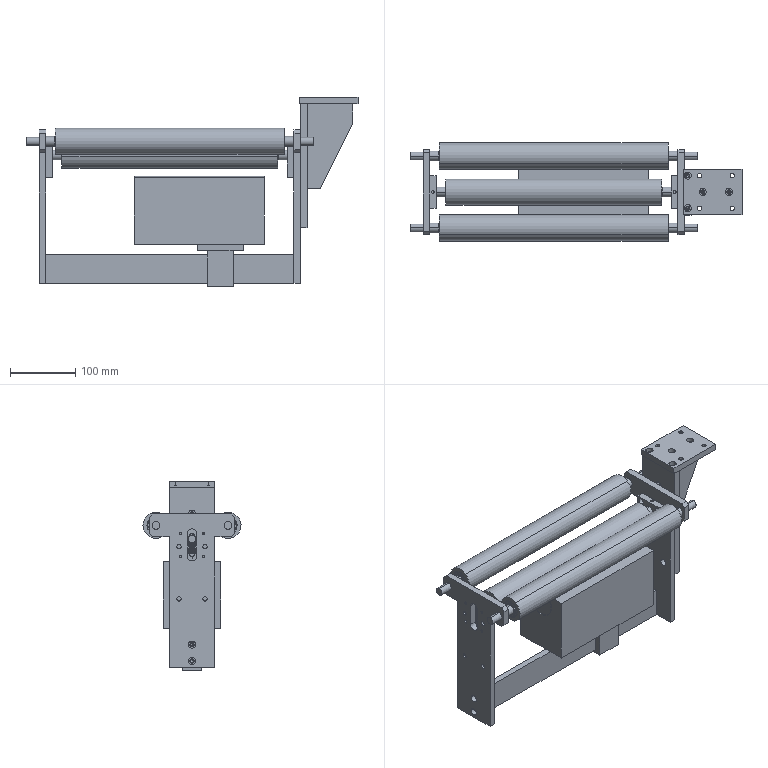Assembly | SolidWorks | mm | 25 component files | 26 solids | 1591 faces | box 508 x 150 x 290 mm | volume 3253189 mm3 | sphere 480 | cylinder 471 | plane 354 | torus 246 | cone 36 | spline 4 | commonest cylinder face diameters 25.2 x48 11 x44 6.6 x44 5 x36 4.2 x32 5.5 x32 15 x30 10 x30
Bill of materials:
01-04MarkingMachineMountingBasePlate | 1 | A3 Steel | Flat rectangular plate with eight round holes through its thickness, in three rows (3-2-3).
01-05MarkingMachineMountingVerticalPlate | 1 | A3 Steel | Thin rectangular bar or plate with six holes through its face and two blind holes drilled into one narrow end face.
01-06MarkingMachineMountingReinforcementPlate | 1 | A3 Steel | Tapered plate: one straight vertical edge, a short parallel section at the top, then an angled edge narrowing toward the bottom. Two blind holes are drilled into the top edge face.
01-07MarkingMachineDrumConnectingPlate1 | 2 | A3 Steel | T-shaped flat plate. The top crossbar has chamfered corners and a large hole at each end. The stem has a central slot with rounded ends near the top, surrounded by small holes, plus further holes lower down.
01-08MarkingMachineDrumConnectingPlate2 | 1 | A3 Steel | Long, solid rectangular bar with two blind holes drilled into one end face.
01-09MarkingMachineIdlerRollerAxis | 2 | A3 Steel | Solid round shaft with stepped ends: a long main section, a short intermediate step, and a smaller-diameter end section at each end.
01-10MarkingMachineIdlerRoller | 2 | A3 Steel | Plain, straight round tube (hollow cylinder) with uniform outside diameter.
01-11CodingRubberRollerMountingPlate | 2 | A3 Steel | Thick, nearly square block with four corner through holes, a central slot with rounded ends, and a cross hole drilled from the top edge face that meets the slot.
01-12MarkingMachinePrintingRollerAxis | 1 | A3 Steel | Long, slender round shaft with reduced-diameter ends. Each end has flat faces and a small hole drilled across it.
01-13MarkingMachinePrintingRoller | 1 | A3 Steel | Plain, straight round tube (hollow cylinder) with uniform outside diameter.
01-14MarkingMachineMountingSeatPlate | 1 | A3 Steel | Rectangular block with a long rectangular opening running through it, and four blind holes near the corners of one face.
01-15MarkingMachineMountingSeatPlate2 | 1 | A3 Steel | Flat rectangular plate with eight round holes through it: four near the corners and four further in, forming a smaller rectangle.
DK1300AInkRollerCoder | 1 | A3 Steel | Rectangular prismatic block with a full-length cylindrical feature running along its long axis just under the top face. The cylinder breaks through the top face and sticks up slightly above it. A thin gap around the cylinder suggests it is a separate rod sitting in a matching through-bore or slot.
GB_T276-94DeepGrooveBallBearing61902-2Z | 6 |  | Annular part shaped like a rolling-element bearing: a concentric outer ring and inner ring with a ring of roughly spherical elements in the annular gap between them, and a plain cylindrical bore.
OuterDiameter10WireDiameter1Height20CompressionSpring | 2 | A3 Steel | Helical coil of round-section wire, shaped like a compression spring, with a flat annular end face and evenly spaced open coils.
Mates:
1. coincident | 01-04MarkingMachineMountingBasePlate-1 face at (-13.91, 2.41, 85) dir (0, 0, -1) | 01-05MarkingMachineMountingVerticalPlate-1 face at (-56.91, -32.59, 85) dir (0, 0, 1)
2. concentric | 01-04MarkingMachineMountingBasePlate-1 face at (-51.91, -22.59, 95) dir (0, 0, 1) r 3.3 | 01-05MarkingMachineMountingVerticalPlate-1 face at (-51.91, -22.59, 85) dir (0, 0, 1) r 2.5
3. concentric | 01-04MarkingMachineMountingBasePlate-1 face at (-51.91, 27.41, 95) dir (0, 0, 1) r 3.3 | 01-05MarkingMachineMountingVerticalPlate-1 face at (-51.91, 27.41, 85) dir (0, 0, 1) r 2.5
4. coincident | 01-04MarkingMachineMountingBasePlate-1 face at (-13.91, 2.41, 85) dir (0, 0, -1) | 01-06MarkingMachineMountingReinforcementPlate-1 face at (-46.91, -2.59, 85) dir (0, 0, 1)
5. coincident | 01-05MarkingMachineMountingVerticalPlate-1 face at (-46.91, 2.41, -10) dir (1, 0, 0) | 01-06MarkingMachineMountingReinforcementPlate-1 face at (-46.91, -2.59, -45) dir (-1, 0, 0)
6. concentric | 01-05MarkingMachineMountingVerticalPlate-1 face at (-56.91, 2.41, -25) dir (-1, 0, 0) r 3.3 | 01-06MarkingMachineMountingReinforcementPlate-1 face at (-46.91, 2.41, -25) dir (-1, 0, 0) r 2.5
7. coincident | 01-05MarkingMachineMountingVerticalPlate-1 face at (-56.91, 2.41, -10) dir (-1, 0, 0) | 01-07MarkingMachineDrumConnectingPlate1-1 face at (-56.91, 2.41, 45) dir (1, 0, 0)
8. concentric | 01-07MarkingMachineDrumConnectingPlate1-1 face at (-66.91, -17.59, -5) dir (-1, 0, 0) r 5.5 | 01-05MarkingMachineMountingVerticalPlate-1 face at (-56.91, -17.59, -5) dir (-1, 0, 0) r 2.5
9. concentric | 01-05MarkingMachineMountingVerticalPlate-1 face at (-56.91, 22.41, -85) dir (-1, 0, 0) r 2.5 | 01-07MarkingMachineDrumConnectingPlate1-1 face at (-66.91, 22.41, -85) dir (-1, 0, 0) r 3.3
10. coincident | 01-07MarkingMachineDrumConnectingPlate1-1 face at (-66.91, 2.41, 45) dir (-1, 0, 0) | 01-08MarkingMachineDrumConnectingPlate2-1 face at (-66.91, -2.59, -190) dir (1, 0, 0)
11. concentric | 01-07MarkingMachineDrumConnectingPlate1-1 face at (-56.91, 2.41, -155) dir (1, 0, 0) r 3.3 | 01-08MarkingMachineDrumConnectingPlate2-1 face at (-66.91, 2.41, -155) dir (1, 0, 0) r 2.5
12. concentric | 01-07MarkingMachineDrumConnectingPlate1-1 face at (-56.91, 2.41, -180) dir (1, 0, 0) r 3.3 | 01-08MarkingMachineDrumConnectingPlate2-1 face at (-66.91, 2.41, -180) dir (1, 0, 0) r 2.5
13. coincident | 01-08MarkingMachineDrumConnectingPlate2-1 face at (-446.91, -2.59, -190) dir (-1, 0, 0) | 01-07MarkingMachineDrumConnectingPlate1-2 face at (-446.91, 2.41, 45) dir (1, 0, 0)
14. concentric | 01-08MarkingMachineDrumConnectingPlate2-1 face at (-446.91, 2.41, -180) dir (-1, 0, 0) r 2.5 | 01-07MarkingMachineDrumConnectingPlate1-2 face at (-456.91, 2.41, -180) dir (-1, 0, 0) r 5.5
15. concentric | 01-08MarkingMachineDrumConnectingPlate2-1 face at (-446.91, 2.41, -155) dir (-1, 0, 0) r 2.5 | 01-07MarkingMachineDrumConnectingPlate1-2 face at (-456.91, 2.41, -155) dir (-1, 0, 0) r 5.5
16. concentric | 01-07MarkingMachineDrumConnectingPlate1-2 face at (-456.91, -52.59, 27.5) dir (1, 0, 0) r 6 | 01-09MarkingMachineIdlerRollerAxis-1 face at (-510.112, -52.59, 27.5) dir (-1, 0, 0) r 7.5
17. coincident | 01-07MarkingMachineDrumConnectingPlate1-2 face at (-446.91, 2.41, 45) dir (1, 0, 0) | 01-09MarkingMachineIdlerRollerAxis-1 face at (-446.91, -46.59, 27.5) dir (-1, 0, 0)
18. concentric | 01-09MarkingMachineIdlerRollerAxis-1 face at (-510.112, -52.59, 27.5) dir (-1, 0, 0) r 7.5 | GB_T276-94DeepGrooveBallBearing61902-2Z-1 face at (-440.831, -52.59, 27.5) dir (-1, 0, 0) r 7.5
19. concentric | 01-09MarkingMachineIdlerRollerAxis-1 face at (-510.112, -52.59, 27.5) dir (-1, 0, 0) r 7.5 | 01-10MarkingMachineIdlerRoller-1 face at (-477.465, -52.59, 27.5) dir (-1, 0, 0) r 20
20. coincident | GB_T276-94DeepGrooveBallBearing61902-2Z-1 face at (-424.91, -39.894, 32.65) dir (1, 0, 0) | 01-10MarkingMachineIdlerRoller-1 face at (-424.91, -40.634, 34.784) dir (-1, 0, 0)
21. concentric | 01-10MarkingMachineIdlerRoller-1 face at (-477.465, -52.59, 27.5) dir (-1, 0, 0) r 20 | GB_T276-94DeepGrooveBallBearing61902-2Z-2 face at (-85.41, -52.59, 27.5) dir (-1, 0, 0) r 14
22. coincident | 01-10MarkingMachineIdlerRoller-1 face at (-88.91, -40.634, 34.784) dir (1, 0, 0) | GB_T276-94DeepGrooveBallBearing61902-2Z-2 face at (-88.91, -39.894, 32.65) dir (-1, 0, 0)
23. coincident | 01-09MarkingMachineIdlerRollerAxis-1 face at (-431.91, -45.44, 27.5) dir (-1, 0, 0) | GB_T276-94DeepGrooveBallBearing61902-2Z-1 face at (-431.91, -44.111, 30.939) dir (-1, 0, 0)
24. concentric | 01-10MarkingMachineIdlerRoller-2 face at (-477.465, 57.41, 27.5) dir (-1, 0, 0) r 12.5 | 01-09MarkingMachineIdlerRollerAxis-2 face at (-510.112, 57.41, 27.5) dir (-1, 0, 0) r 7.5
25. concentric | 01-09MarkingMachineIdlerRollerAxis-2 face at (-510.112, 57.41, 27.5) dir (-1, 0, 0) r 7.5 | GB_T276-94DeepGrooveBallBearing61902-2Z-3 face at (-85.41, 57.41, 27.5) dir (-1, 0, 0) r 14
26. coincident | 01-10MarkingMachineIdlerRoller-2 face at (-88.91, 68.746, 35.716) dir (1, 0, 0) | GB_T276-94DeepGrooveBallBearing61902-2Z-3 edge at (-88.91, 57.41, 27.5) dir (-1, 0, 0) r 13.7
27. coincident | 01-10MarkingMachineIdlerRoller-2 face at (-424.91, 68.746, 35.716) dir (-1, 0, 0) | GB_T276-94DeepGrooveBallBearing61902-2Z-4 face at (-424.91, 65.889, 30.939) dir (1, 0, 0)
28. concentric | 01-10MarkingMachineIdlerRoller-2 face at (-477.465, 57.41, 27.5) dir (-1, 0, 0) r 14 | GB_T276-94DeepGrooveBallBearing61902-2Z-4 face at (-428.41, 57.41, 27.5) dir (-1, 0, 0) r 14
29. coincident | 01-09MarkingMachineIdlerRollerAxis-2 face at (-81.91, 64.56, 27.5) dir (1, 0, 0) | GB_T276-94DeepGrooveBallBearing61902-2Z-3 face at (-81.91, 65.889, 30.939) dir (1, 0, 0)
30. concentric | 01-07MarkingMachineDrumConnectingPlate1-1 face at (-56.91, 57.41, 27.5) dir (-1, 0, 0) r 6 | 01-09MarkingMachineIdlerRollerAxis-2 face at (-510.112, 57.41, 27.5) dir (-1, 0, 0) r 7.5
31. coincident | 01-09MarkingMachineIdlerRollerAxis-1 face at (-36.91, -52.59, 27.5) dir (1, 0, 0) | 01-09MarkingMachineIdlerRollerAxis-2 face at (-36.91, 57.41, 27.5) dir (1, 0, 0)
32. coincident | 01-07MarkingMachineDrumConnectingPlate1-2 face at (-446.91, 2.41, 45) dir (1, 0, 0) | 01-11CodingRubberRollerMountingPlate-1 face at (-446.91, 2.41, -2.5) dir (-1, 0, 0)
33. slot | 01-12MarkingMachinePrintingRollerAxis-1 face at (-510.112, 2.41, 6.568) dir (-1, 0, 0) r 7.5 | 01-11CodingRubberRollerMountingPlate-1 face at (-446.91, 2.41, -15) dir (1, 0, 0) r 5
34. coincident | 01-11CodingRubberRollerMountingPlate-1 face at (-436.91, 2.41, -2.5) dir (1, 0, 0) | 01-12MarkingMachinePrintingRollerAxis-1 face at (-436.91, -3.59, 6.568) dir (-1, 0, 0)
35. coincident | 01-07MarkingMachineDrumConnectingPlate1-1 face at (-66.91, 2.41, 45) dir (-1, 0, 0) | 01-11CodingRubberRollerMountingPlate-2 face at (-66.91, 2.41, -2.5) dir (1, 0, 0)
36. concentric | 01-07MarkingMachineDrumConnectingPlate1-1 face at (-56.91, 19.91, -20) dir (1, 0, 0) r 2.1 | 01-11CodingRubberRollerMountingPlate-2 face at (-76.91, 19.91, -20) dir (-1, 0, 0) r 2.75
37. concentric | 01-07MarkingMachineDrumConnectingPlate1-1 face at (-56.91, -15.09, 15) dir (1, 0, 0) r 2.1 | 01-11CodingRubberRollerMountingPlate-2 face at (-76.91, -15.09, 15) dir (-1, 0, 0) r 2.75
38. coincident | 01-11CodingRubberRollerMountingPlate-1 face at (-446.91, -2.59, -15) dir (0, 1, 0) | 01-12MarkingMachinePrintingRollerAxis-1 face at (-446.91, -2.59, 14.068) dir (0, -1, 0)
39. concentric | 01-07MarkingMachineDrumConnectingPlate1-2 face at (-456.91, -15.09, 15) dir (-1, 0, 0) r 2.1 | 01-11CodingRubberRollerMountingPlate-1 face at (-436.91, -15.09, 15) dir (1, 0, 0) r 2.75
40. concentric | 01-07MarkingMachineDrumConnectingPlate1-2 face at (-456.91, 19.91, -20) dir (-1, 0, 0) r 2.1 | 01-11CodingRubberRollerMountingPlate-1 face at (-436.91, 19.91, -20) dir (1, 0, 0) r 5
41. concentric | 01-11CodingRubberRollerMountingPlate-1 face at (-441.91, 2.41, 22.501) dir (0, 0, -1) r 3.432 | OuterDiameter10WireDiameter1Height20CompressionSpring-1 sketch segment at (-441.91, 2.41, -15.758) dir (0, 0, 1) r 4.25
42. distance | OuterDiameter10WireDiameter1Height20CompressionSpring-1 face at (-450.41, -2.59, -15) dir (0, 0, -1) | 01-11CodingRubberRollerMountingPlate-1 face at (-436.91, 27.41, -27.5) dir (0, 0, -1)
43. concentric | 01-11CodingRubberRollerMountingPlate-2 face at (-71.91, 2.41, 22.501) dir (0, 0, -1) r 3.432 | OuterDiameter10WireDiameter1Height20CompressionSpring-2 sketch segment at (-71.91, 2.41, -15.758) dir (0, 0, 1) r 4.25
44. distance | OuterDiameter10WireDiameter1Height20CompressionSpring-2 face at (-76.451, -6.343, -15) dir (0, 0, -1) | 01-11CodingRubberRollerMountingPlate-2 face at (-76.91, -22.59, -27.5) dir (0, 0, -1)
45. concentric | 01-12MarkingMachinePrintingRollerAxis-1 face at (-510.112, 2.41, 6.568) dir (-1, 0, 0) r 7.5 | 01-13MarkingMachinePrintingRoller-1 face at (-477.465, 2.41, 6.568) dir (-1, 0, 0) r 20
46. concentric | 01-13MarkingMachinePrintingRoller-1 face at (-477.465, 2.41, 6.568) dir (-1, 0, 0) r 14 | GB_T276-94DeepGrooveBallBearing61902-2Z-5 face at (-418.41, 2.41, 6.568) dir (-1, 0, 0) r 14
47. coincident | 01-13MarkingMachinePrintingRoller-1 face at (-414.91, 4.237, -7.312) dir (-1, 0, 0) | GB_T276-94DeepGrooveBallBearing61902-2Z-5 face at (-414.91, 10.889, 10.007) dir (1, 0, 0)
48. coincident | 01-12MarkingMachinePrintingRollerAxis-1 face at (-421.91, -4.74, 6.568) dir (-1, 0, 0) | GB_T276-94DeepGrooveBallBearing61902-2Z-5 face at (-421.91, 10.889, 10.007) dir (-1, 0, 0)
49. coincident | 01-13MarkingMachinePrintingRoller-1 face at (-98.91, 4.237, -7.312) dir (1, 0, 0) | GB_T276-94DeepGrooveBallBearing61902-2Z-6 face at (-98.91, 10.889, 10.007) dir (-1, 0, 0)
50. concentric | 01-13MarkingMachinePrintingRoller-1 face at (-477.465, 2.41, 6.568) dir (-1, 0, 0) r 14 | GB_T276-94DeepGrooveBallBearing61902-2Z-6 face at (-95.41, 2.41, 6.568) dir (-1, 0, 0) r 14
51. coincident | 01-08MarkingMachineDrumConnectingPlate2-1 face at (-446.91, -2.59, -145) dir (0, 0, 1) | 01-14MarkingMachineMountingSeatPlate-1 face at (-159.532, -2.59, -145) dir (0, 0, -1)
52. coincident | 01-08MarkingMachineDrumConnectingPlate2-1 face at (-256.91, -2.59, -167.5) dir (0, -1, 0) | 01-14MarkingMachineMountingSeatPlate-1 face at (-159.532, -2.59, -145) dir (0, 1, 0)
53. coincident | 01-14MarkingMachineMountingSeatPlate-1 face at (-159.532, -12.59, -140) dir (0, 0, 1) | 01-15MarkingMachineMountingSeatPlate2-1 face at (-179.532, 2.41, -140) dir (0, 0, -1)
54. concentric | 01-14MarkingMachineMountingSeatPlate-1 face at (-194.532, -7.59, -140) dir (0, 0, 1) r 2.1 | 01-15MarkingMachineMountingSeatPlate2-1 face at (-194.532, -7.59, -130) dir (0, 0, 1) r 2.75
55. concentric | 01-14MarkingMachineMountingSeatPlate-1 face at (-164.532, 12.41, -140) dir (0, 0, 1) r 2.1 | 01-15MarkingMachineMountingSeatPlate2-1 face at (-164.532, 12.41, -130) dir (0, 0, 1) r 5
56. coincident | 01-15MarkingMachineMountingSeatPlate2-1 face at (-179.532, 2.41, -130) dir (0, 0, 1) | DK1300AInkRollerCoder-1 face at (-212.032, 2.41, -130) dir (0, 0, -1)
57. concentric | 01-15MarkingMachineMountingSeatPlate2-1 face at (-152.532, 18.41, -140) dir (0, 0, -1) r 2.75 | DK1300AInkRollerCoder-1 face at (-152.532, 18.41, -130) dir (0, 0, -1) r 2.5
58. concentric | 01-15MarkingMachineMountingSeatPlate2-1 edge at (-152.532, -13.59, -130) dir (0, 0, -1) r 2.75 | DK1300AInkRollerCoder-1 edge at (-152.532, -13.59, -130) dir (0, 0, -1) r 2.5